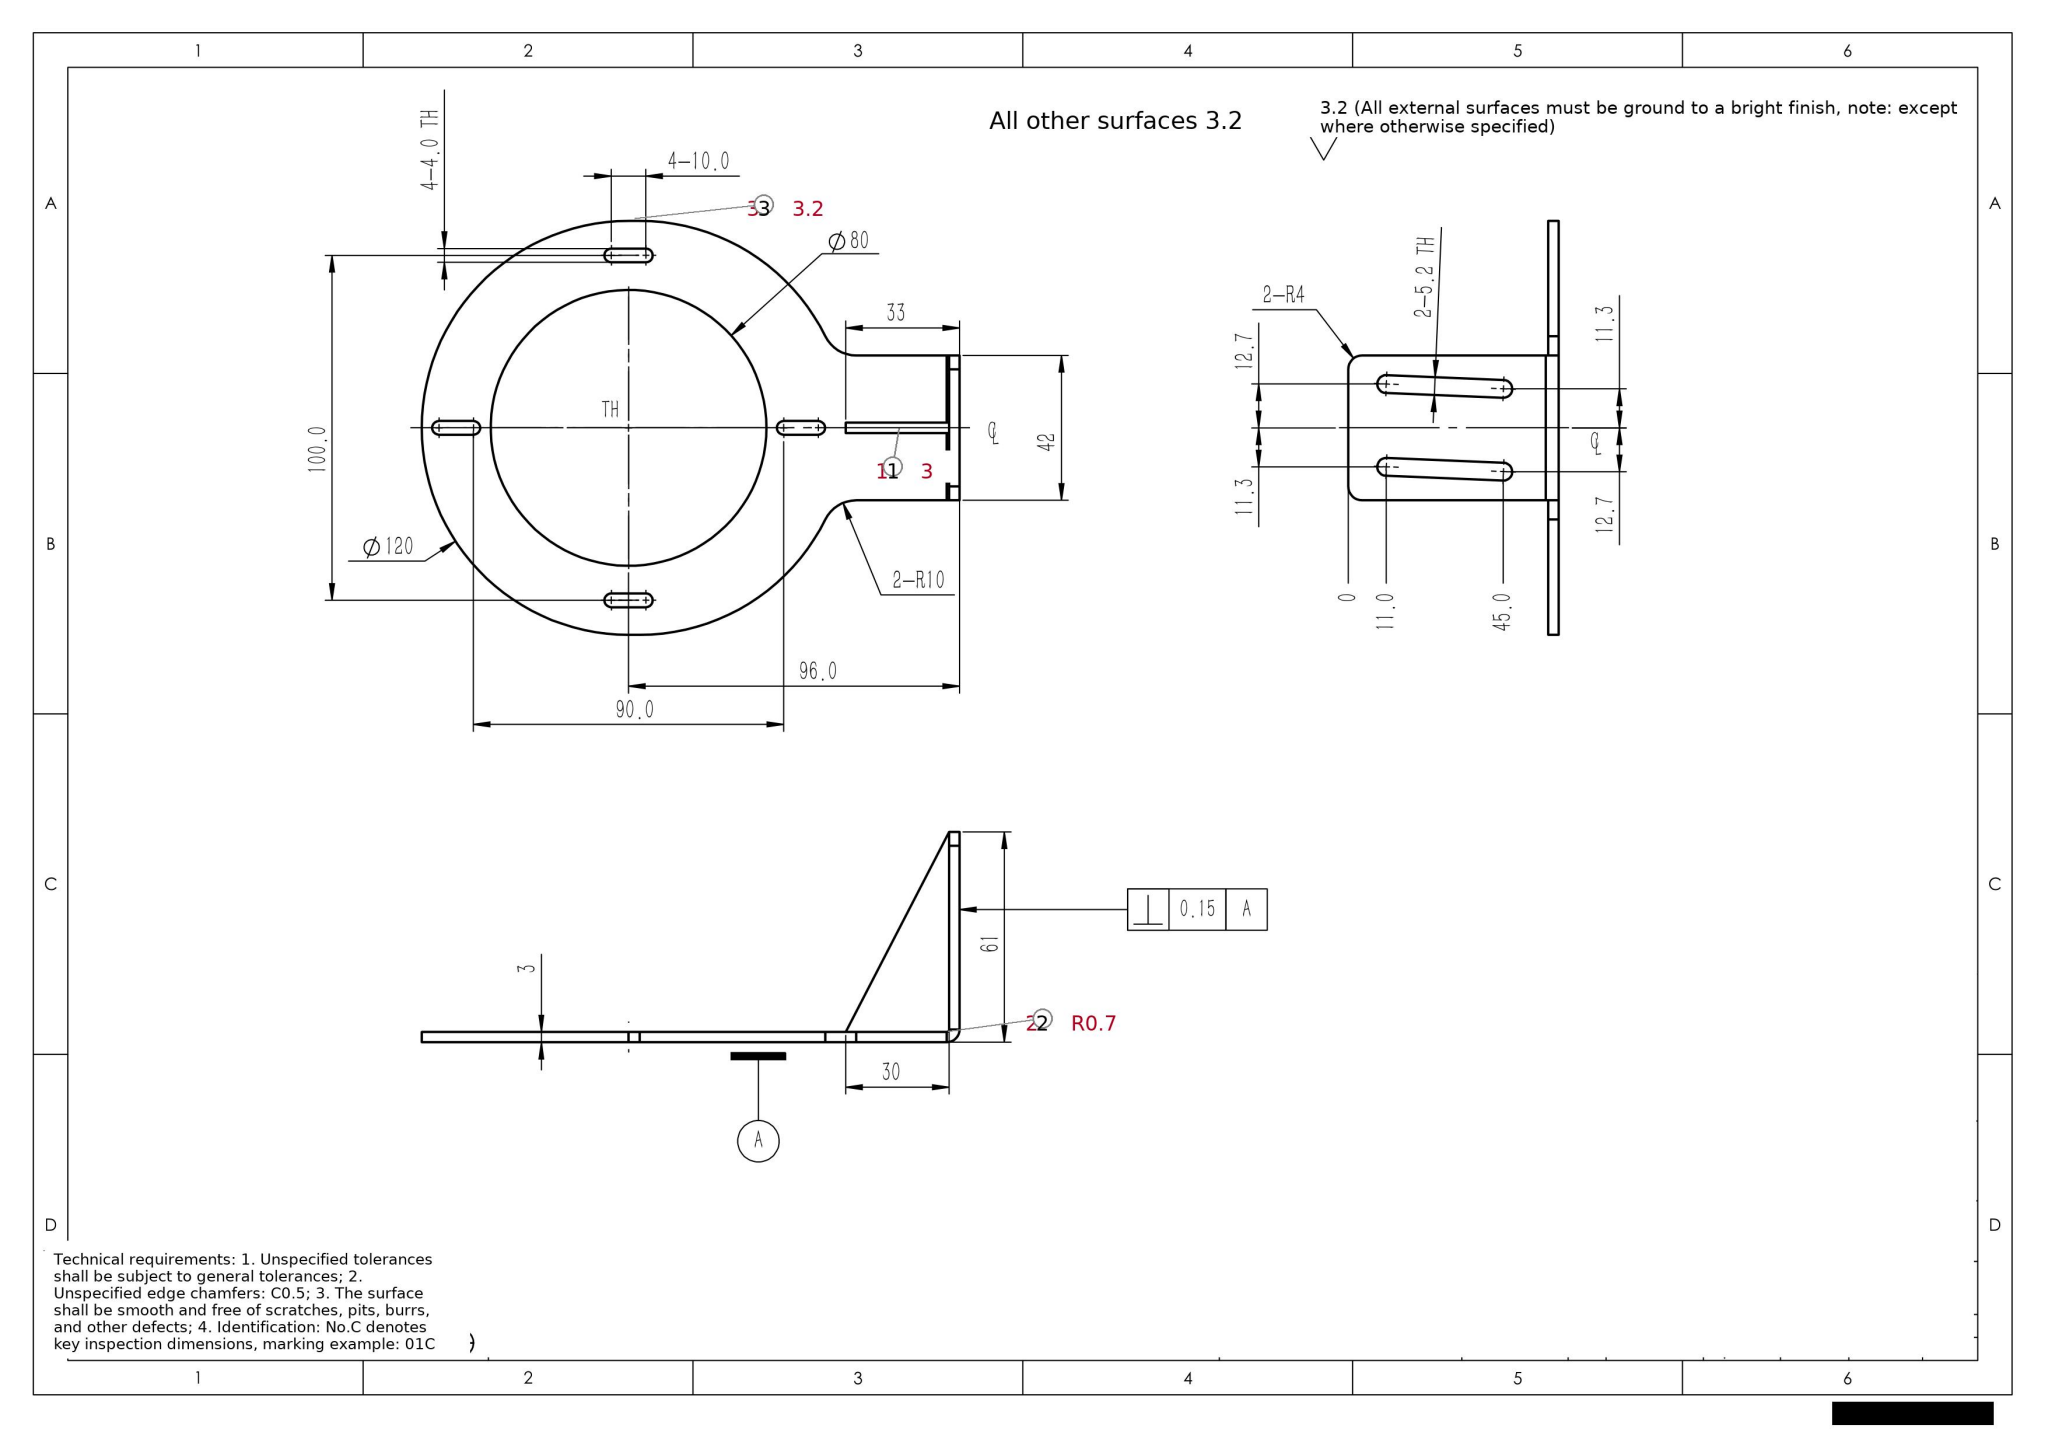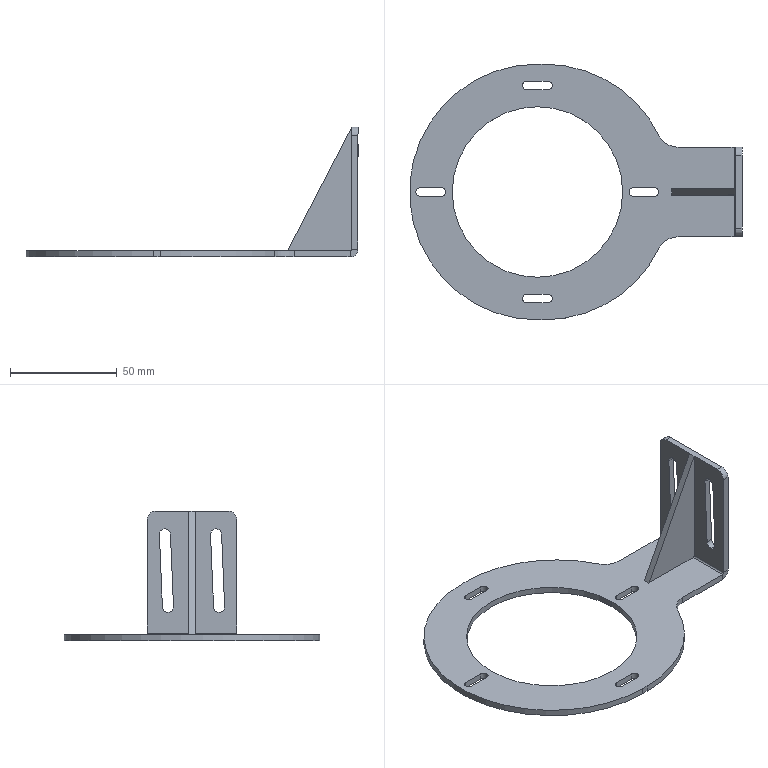Part | SolidWorks | mm | 1 solid | 59 faces | box 156 x 120 x 61 mm | volume 32301 mm3 | cylinder 30 | plane 29 | commonest cylinder face diameters 4 x12 5.2 x6 120 x3 80 x2 1.473 x2 20 x2 8 x2 7.473 x1